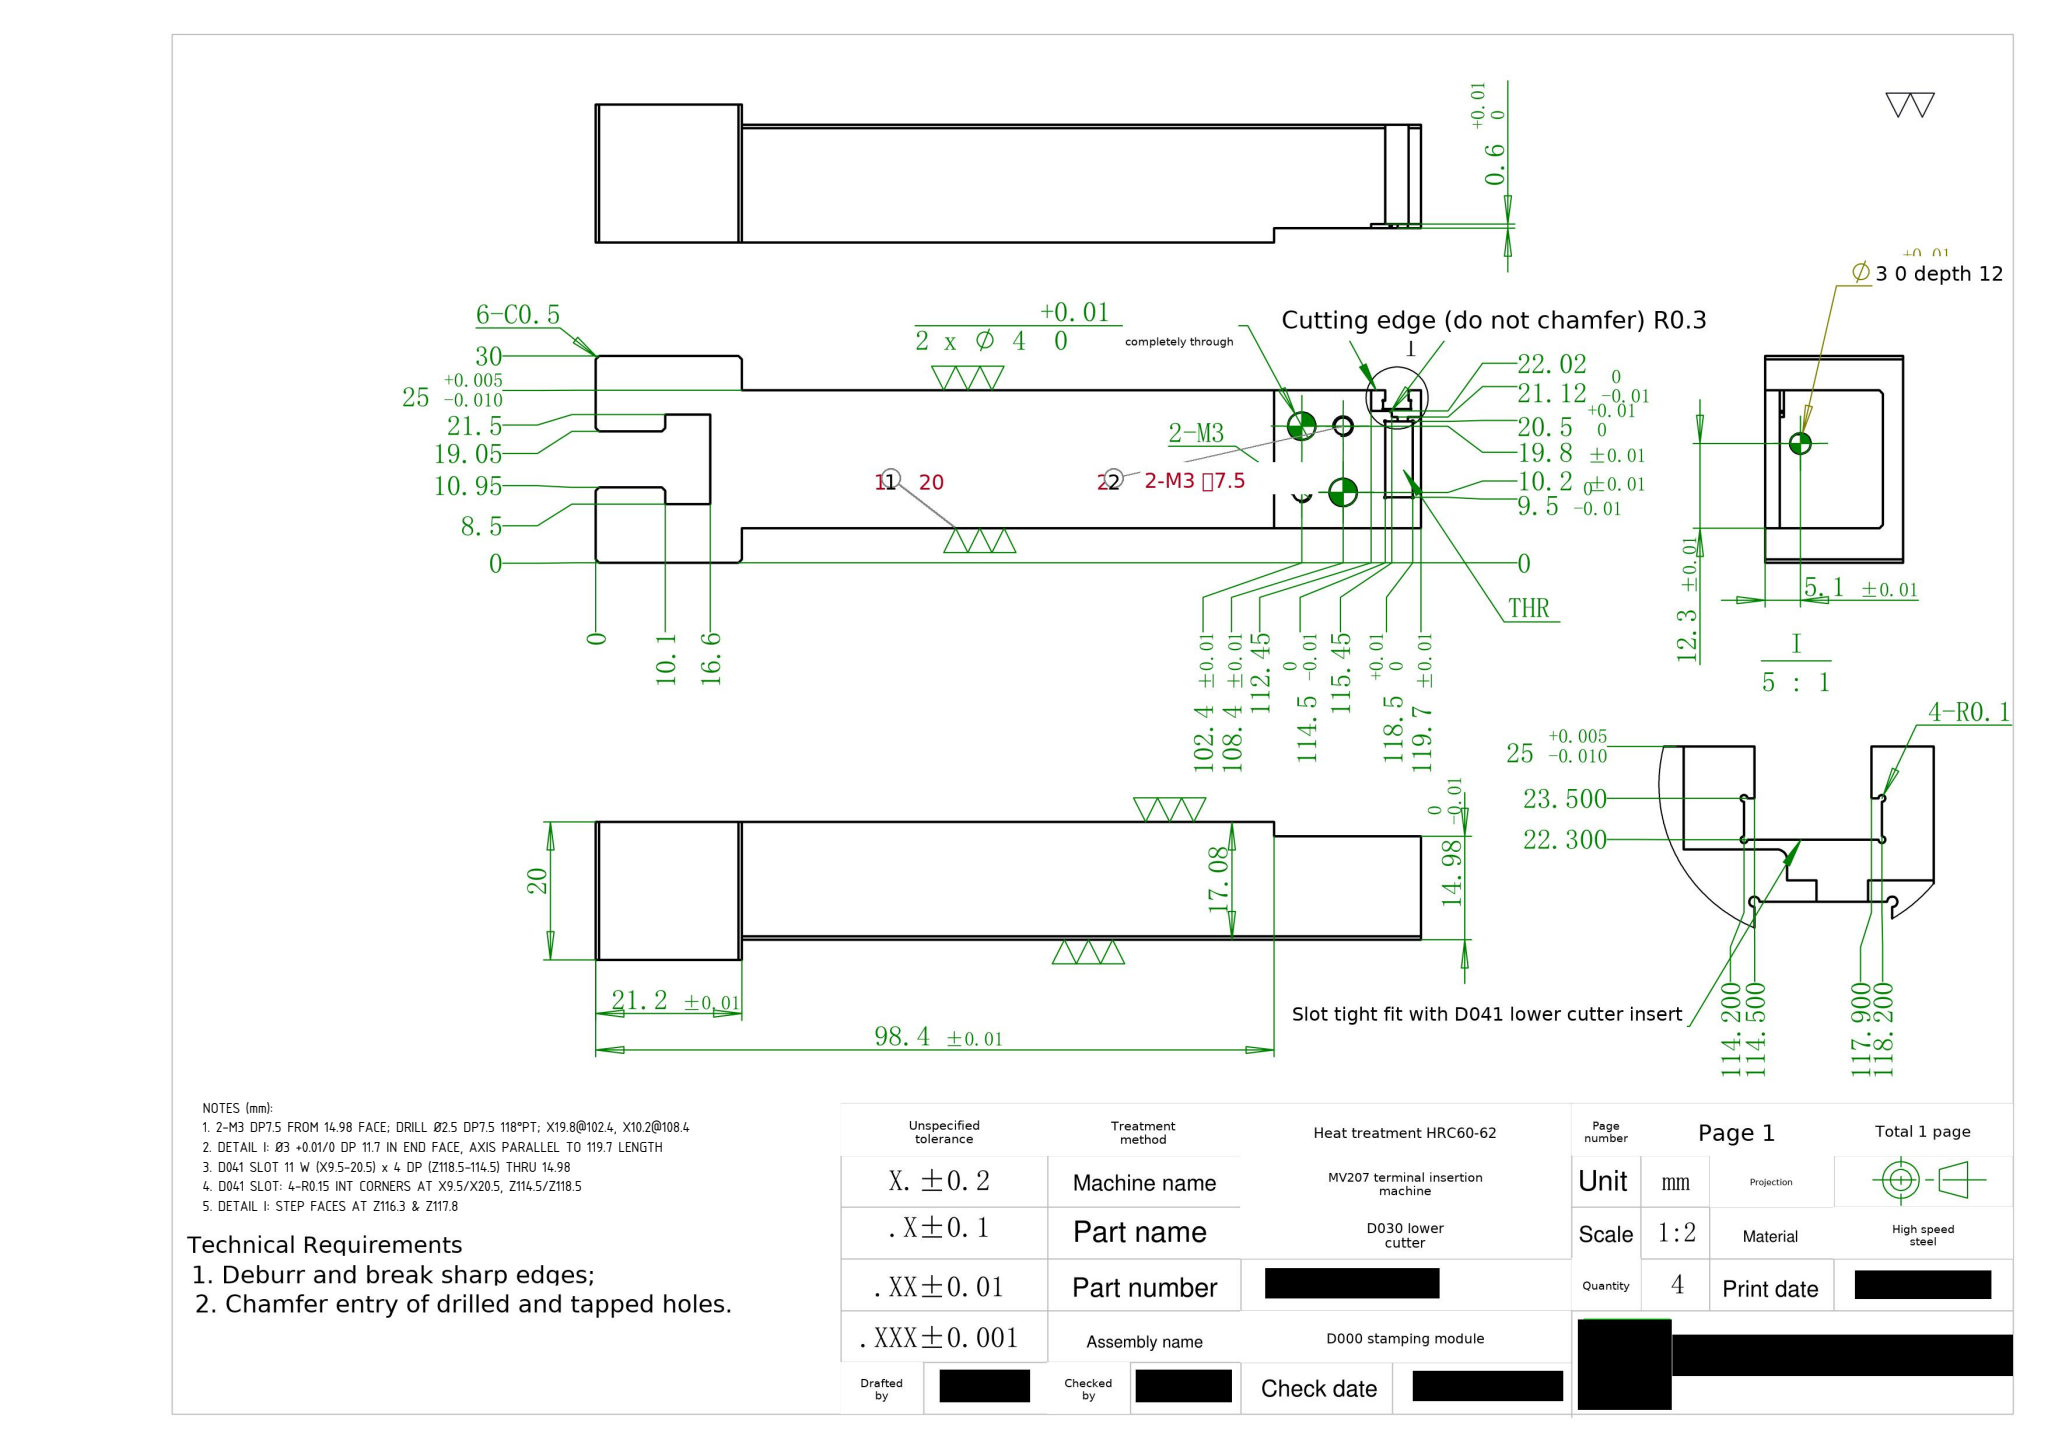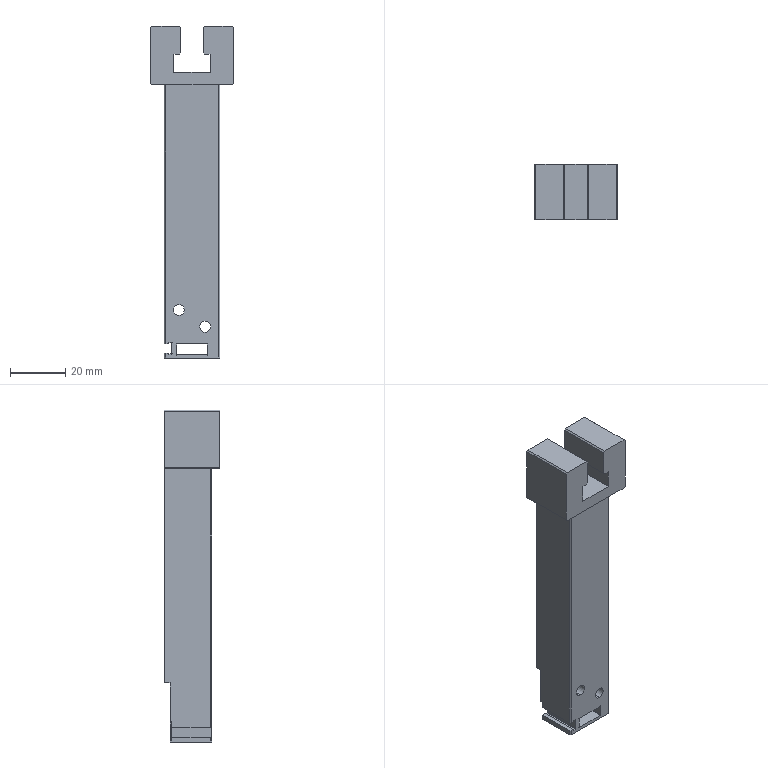Part | SolidWorks | mm | 1 solid | 81 faces | box 30 x 20 x 119.7 mm | volume 40774 mm3 | plane 52 | cylinder 25 | cone 4 | commonest cylinder face diameters 0.2 x6 0.3 x6 3 x4 4 x4 2.5 x4 0.6 x1
Drawing notes:
2-M3 DP7.5 FROM 14.98 FACE; DRILL Ø2.5 DP7.5 118°PT; X19.8@102.4, X10.2@108.4 | from the solid: cyl Ø2.5 axis Y len 7.5 at (x10.2,z11.3)->108.4 & (x19.8,z17.3)->102.4; cones 118° ref dia 2.5; thk y2.92-17.9=14.98
DETAIL I: Ø3 +0.01/0 DP 11.7 IN END FACE, AXIS PARALLEL TO 119.7 LENGTH | from the solid: cyl Ø3.0 axis Z at (12.7,14.9), segs 6.5+1.2 broken by slot z1.2-5.2, end z-plane 11.7
D041 SLOT 11 W (X9.5-20.5) x 4 DP (Z118.5-114.5) THRU 14.98 | from the solid: corner cyls at x9.5 & 20.5, z1.2 & 5.2, len 14.98; 119.7-1.2=118.5, 119.7-5.2=114.5
D041 SLOT: 4-R0.15 INT CORNERS AT X9.5/X20.5, Z114.5/Z118.5 | from the solid: 4x cyl Ø0.3 axis Y at x9.5 & 20.5, z1.2 & 5.2, len 14.98 -> R0.15
DETAIL I: STEP FACES AT Z116.3 & Z117.8 | from the solid: axis_planes normal z at 3.4 and 1.9; 119.7-3.4=116.3, 119.7-1.9=117.8
build123d program:
from build123d import *

# Parameters (mm, degrees)
SKETCH1_W                = 20
SKETCH1_H                = 115
BOSS_EXTRUDE1_DEPTH      = 14.98
CUT_EXTRUDE2_DEPTH       = 0.6
FILLET1_R                = 0.3
SKETCH4_W                = 10
SKETCH4_H                = 14.98
BOSS_EXTRUDE2_DEPTH      = 2
CUT_EXTRUDE3_DEPTH       = 61.619
SKETCH12_W               = 10
SKETCH12_H               = 14.98
CUT_EXTRUDE7_DEPTH       = 2
M3_TAPPED_HOLE1_D        = 2.5
M3_TAPPED_HOLE1_DEPTH    = 7.5
M3_TAPPED_HOLE1_TIP      = 0.7511
F_4_0_4_DIAMETER_HOLE1_D = 4
SKETCH18_W               = 11
SKETCH18_H               = 4
CUT_EXTRUDE9_DEPTH       = 61.255
SKETCH20_R               = 1.5
CUT_EXTRUDE10_DEPTH      = 12
SKETCH22_W               = 5.95
SKETCH22_H               = 14.98
BOSS_EXTRUDE4_DEPTH      = 5
BOSS_EXTRUDE5_DEPTH      = 2.1
BOSS_EXTRUDE6_DEPTH      = 2.92
CHAMFER2_SIZE            = 0.5
CHAMFER3_SIZE            = 0.5
SKETCH26_R               = 0.15
CUT_EXTRUDE13_DEPTH      = 66.777
CUT_EXTRUDE14_DEPTH      = 0.3
CUT_EXTRUDE15_DEPTH      = 66.617
SKETCH29_R               = 0.1
CUT_EXTRUDE16_DEPTH      = 66.617
SKETCH30_W               = 0.62
SKETCH30_H               = 1.5
CUT_EXTRUDE17_DEPTH      = 0.6
SKETCH31_W               = 21.2
SKETCH31_H               = 20
BOSS_EXTRUDE7_DEPTH      = 5
CHAMFER5_SIZE            = 0.5


with BuildPart() as part:
    # Sketch1 → Boss-Extrude1 (new body)
    with BuildSketch(Plane(origin=(0, 0, 0), x_dir=(1, 0, 0), z_dir=(0, 1, 0))):
        Rectangle(SKETCH1_W, SKETCH1_H)
    extrude(amount=BOSS_EXTRUDE1_DEPTH)

    # Sketch3 → Cut-Extrude2 (cut)
    with BuildSketch(Plane(origin=(0, 14.98, 0), x_dir=(1, 0, 0), z_dir=(0, 1, 0))):
        Polygon((-6.12, 57.5), (-6.12, 52.95), (-7.02, 52.95), (-7.02, 49.95), (-10, 49.95), (-10, 57.5), align=None)
    extrude(amount=-CUT_EXTRUDE2_DEPTH, mode=Mode.SUBTRACT)

    # Fillet1
    fillet1_edges = [part.edges().sort_by_distance(p)[0] for p in [
        (-7.02, 14.68, -52.95),
    ]]
    fillet(fillet1_edges, radius=FILLET1_R)

    # Sketch4 → Boss-Extrude2 (add)
    with BuildSketch(Plane(origin=(10, 0, 0), x_dir=(0, 0, -1), z_dir=(1, 0, 0))):
        with Locations((52.5, 7.49)):
            Rectangle(SKETCH4_W, SKETCH4_H)
    extrude(amount=BOSS_EXTRUDE2_DEPTH)

    # Sketch2 → Cut-Extrude3 (cut, through all)
    with BuildSketch(Plane(origin=(0, 14.98, 0), x_dir=(1, 0, 0), z_dir=(0, 1, 0))):
        Polygon((-4.05, -57.5), (-4.05, -52.4), (-6.5, -52.4), (-6.5, -45.9), (6.5, -45.9), (6.5, -52.4), (4.05, -52.4), (4.05, -57.5), align=None)
    extrude(amount=-CUT_EXTRUDE3_DEPTH, mode=Mode.SUBTRACT)

    # Sketch12 → Cut-Extrude7 (cut)
    with BuildSketch(Plane(origin=(12, 0, 0), x_dir=(0, 0, -1), z_dir=(1, 0, 0))):
        with Locations((52.5, 7.49)):
            Rectangle(SKETCH12_W, SKETCH12_H)
    extrude(amount=-CUT_EXTRUDE7_DEPTH, mode=Mode.SUBTRACT)

    # M3 Tapped Hole1
    with Locations(Plane(origin=(0, 14.98, 0), x_dir=(1, 0, 0), z_dir=(0, 1, 0))):
        with Locations((4.8, 39.9), (-4.8, 45.9)):
            Hole(M3_TAPPED_HOLE1_D / 2, depth=M3_TAPPED_HOLE1_DEPTH)
            with Locations((0, 0, -(M3_TAPPED_HOLE1_DEPTH + M3_TAPPED_HOLE1_TIP / 2))):  # 118° drill point
                Cone(0, M3_TAPPED_HOLE1_D / 2, M3_TAPPED_HOLE1_TIP, mode=Mode.SUBTRACT)

    # 4.0 _4_ Diameter Hole1 (through all)
    with Locations(Plane(origin=(0, 14.98, 0), x_dir=(1, 0, 0), z_dir=(0, 1, 0))):
        with Locations((4.8, 45.9), (-4.8, 39.9)):
            Hole(F_4_0_4_DIAMETER_HOLE1_D / 2)

    # Sketch18 → Cut-Extrude9 (cut, through all)
    with BuildSketch(Plane(origin=(0, 14.98, 0), x_dir=(1, 0, 0), z_dir=(0, 1, 0))):
        with Locations((0, 54)):
            Rectangle(SKETCH18_W, SKETCH18_H)
    extrude(amount=-CUT_EXTRUDE9_DEPTH, mode=Mode.SUBTRACT)

    # Sketch20 → Cut-Extrude10 (cut)
    with BuildSketch(Plane(origin=(0, 0, -57.5), x_dir=(-1, 0, 0), z_dir=(0, 0, -1))):
        with Locations((2.3, 11.98)):
            Circle(SKETCH20_R)
    extrude(amount=-CUT_EXTRUDE10_DEPTH, mode=Mode.SUBTRACT)

    # Sketch22 → Boss-Extrude4 (add)
    with BuildSketch(Plane.XY.offset(57.5)):
        with Locations((7.025, 7.49)):
            Rectangle(SKETCH22_W, SKETCH22_H)
        with Locations((-7.025, 7.49)):
            Rectangle(SKETCH22_W, SKETCH22_H)
    extrude(amount=BOSS_EXTRUDE4_DEPTH)

    # Sketch23 → Boss-Extrude5 (add)
    with BuildSketch(Plane(origin=(0, 14.98, 0), x_dir=(1, 0, 0), z_dir=(0, 1, 0))):
        Polygon((-10, 35.9), (10, 35.9), (10, -62.5), (4.05, -62.5), (4.05, -52.4), (6.5, -52.4), (6.5, -45.9), (-6.5, -45.9), (-6.5, -52.4), (-4.05, -52.4), (-4.05, -62.5), (-10, -62.5), align=None)
    extrude(amount=BOSS_EXTRUDE5_DEPTH)

    # Sketch25 → Boss-Extrude6 (add)
    with BuildSketch(Plane.XZ):
        Polygon((10, 41.3), (-10, 41.3), (-10, 62.5), (-4.05, 62.5), (-4.05, 52.4), (-6.5, 52.4), (-6.5, 45.9), (6.5, 45.9), (6.5, 52.4), (4.05, 52.4), (4.05, 62.5), (10, 62.5), align=None)
    extrude(amount=BOSS_EXTRUDE6_DEPTH)

    # Chamfer2
    chamfer2_edges = [part.edges().sort_by_distance(p)[0] for p in [
        (4.05, 7.08, 62.5),
        (-4.05, 7.08, 62.5),
        (-4.05, 7.08, 52.4),
        (4.05, 7.08, 52.4),
    ]]
    chamfer(chamfer2_edges, length=CHAMFER2_SIZE)

    # Chamfer3
    chamfer3_edges = [part.edges().sort_by_distance(p)[0] for p in [
        (-10, 0, -8.1),
        (10, 0, -8.1),
    ]]
    chamfer(chamfer3_edges, length=CHAMFER3_SIZE)

    # Sketch26 → Cut-Extrude13 (cut, through all)
    with BuildSketch(Plane(origin=(0, 14.98, 0), x_dir=(1, 0, 0), z_dir=(0, 1, 0))):
        with Locations((5.5, 56)):
            Circle(SKETCH26_R)
        with Locations((5.5, 52)):
            Circle(SKETCH26_R)
        with Locations((-5.5, 52)):
            Circle(SKETCH26_R)
        with Locations((-5.5, 56)):
            Circle(SKETCH26_R)
    extrude(amount=-CUT_EXTRUDE13_DEPTH, mode=Mode.SUBTRACT)

    # Sketch27 → Cut-Extrude14 (cut)
    with BuildSketch(Plane(origin=(0, 0, -57.5), x_dir=(-1, 0, 0), z_dir=(0, 0, -1))):
        Polygon((-10, 14.98), (-10, 0.5), (-9.5, 0), (9.5, 0), (10, 0.5), (10, 14.38), (6.12, 14.38), (6.12, 14.98), align=None)
    extrude(amount=-CUT_EXTRUDE14_DEPTH, mode=Mode.SUBTRACT)

    # Sketch28 → Cut-Extrude15 (cut, through all)
    with BuildSketch(Plane(origin=(0, 14.38, 0), x_dir=(1, 0, 0), z_dir=(0, 1, 0))):
        Polygon((-10, 52), (-8.5, 52), (-8.5, 51.7), (-7.3, 51.7), (-7.3, 55.7), (-8.5, 55.7), (-8.5, 55.4), (-10, 55.4), align=None)
    extrude(amount=-CUT_EXTRUDE15_DEPTH, mode=Mode.SUBTRACT)

    # Sketch29 → Cut-Extrude16 (cut, through all)
    with BuildSketch(Plane(origin=(0, 14.38, 0), x_dir=(1, 0, 0), z_dir=(0, 1, 0))):
        with Locations((-8.5, 51.7)):
            Circle(SKETCH29_R)
        with Locations((-7.3, 51.7)):
            Circle(SKETCH29_R)
        with Locations((-7.3, 55.7)):
            Circle(SKETCH29_R)
        with Locations((-8.5, 55.7)):
            Circle(SKETCH29_R)
    extrude(amount=-CUT_EXTRUDE16_DEPTH, mode=Mode.SUBTRACT)

    # Sketch30 → Cut-Extrude17 (cut)
    with BuildSketch(Plane(origin=(0, 14.98, 0), x_dir=(1, 0, 0), z_dir=(0, 1, 0))):
        with Locations((-5.81, 54.55)):
            Rectangle(SKETCH30_W, SKETCH30_H)
    extrude(amount=-CUT_EXTRUDE17_DEPTH, mode=Mode.SUBTRACT)

    # Sketch31 → Boss-Extrude7 (add)
    with BuildSketch(Plane(origin=(10, 0, 0), x_dir=(0, 0, -1), z_dir=(1, 0, 0))):
        with Locations((-51.9, 7.08)):
            Rectangle(SKETCH31_W, SKETCH31_H)
    boss_extrude7 = extrude(amount=BOSS_EXTRUDE7_DEPTH)

    # Mirror1: Boss-Extrude7 across plane
    add(boss_extrude7.mirror(Plane(origin=(0, 0, 0), x_dir=(0, 0, 1), z_dir=(1, 0, 0))))

    # Chamfer5
    chamfer5_edges = [part.edges().sort_by_distance(p)[0] for p in [
        (-15, 7.08, 62.5),
        (-15, 7.08, 41.3),
        (15, 7.08, 41.3),
        (15, 7.08, 62.5),
    ]]
    chamfer(chamfer5_edges, length=CHAMFER5_SIZE)


solid = part.part